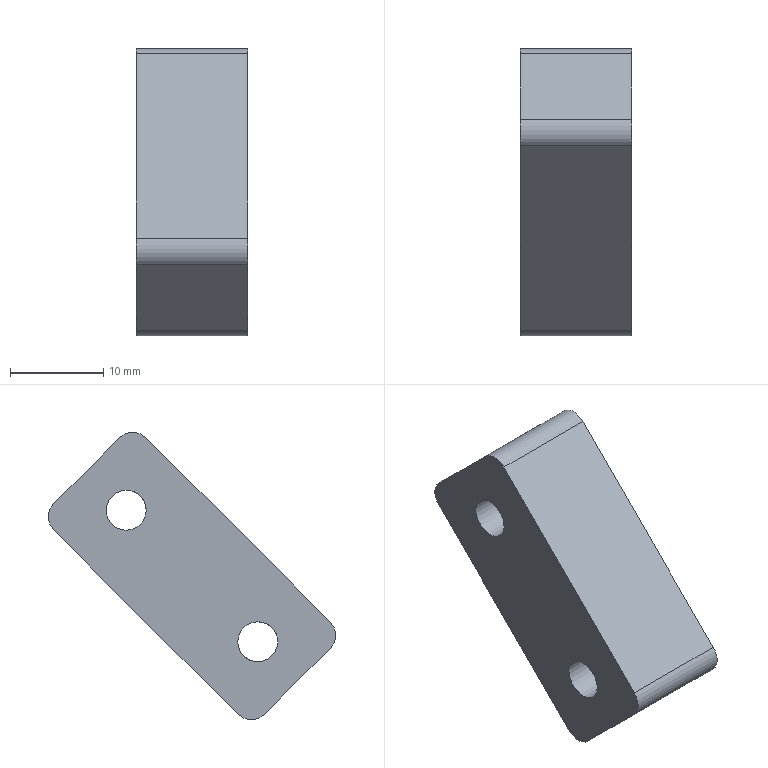Component | NX | SPACER_BLOCK_2 | 1 solid | 16 faces | volume 4670 mm3 | cylinder 8 | plane 8 | commonest cylinder face diameters 4 x4 4.3 x2 8.3 x2